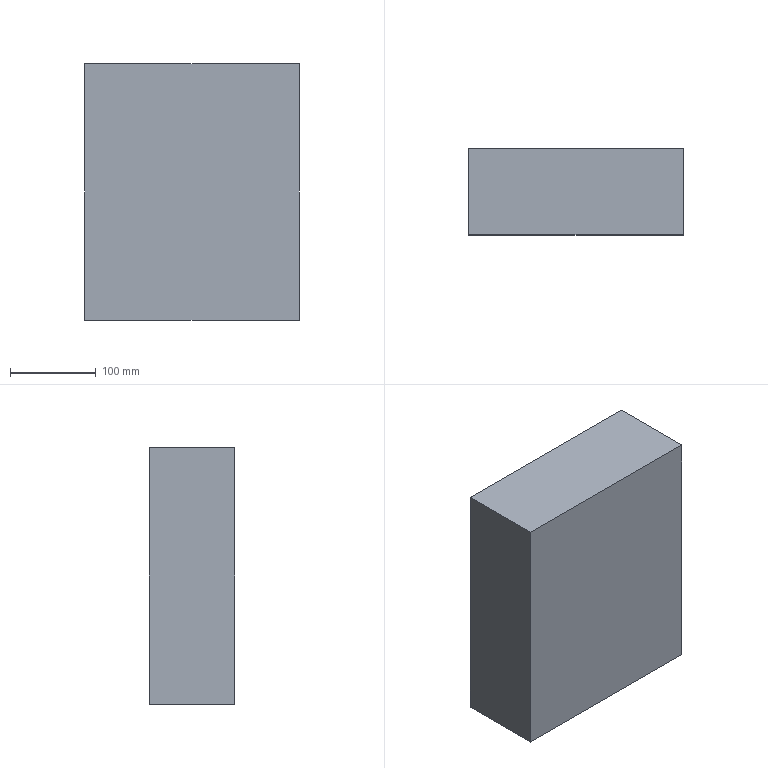Component | SolidWorks | InsectCollectionBox-1 | 1 solid | 11 faces | box 250 x 100 x 300 mm | volume 274138 mm3 | plane 11
build123d program:
from build123d import *

# Parameters (mm, degrees)
SKETCH1_W           = 300
SKETCH1_H           = 250
BOSS_EXTRUDE1_DEPTH = 100
SHELL1_T            = -1.5


with BuildPart() as part:
    # Sketch1 → Boss-Extrude1 (new body)
    with BuildSketch(Plane(origin=(0, 0, 0), x_dir=(1, 0, 0), z_dir=(0, 1, 0))):
        Rectangle(SKETCH1_W, SKETCH1_H)
    extrude(amount=BOSS_EXTRUDE1_DEPTH)

    # Shell1
    shell1_openings = [part.faces().sort_by_distance(p)[0] for p in [
        (0, 100, 0),
    ]]
    offset(amount=SHELL1_T, openings=shell1_openings, kind=Kind.INTERSECTION)


solid = part.part

# Placed as in the assembly
solid = solid.moved(Location((173.5, 1.5, 0), (0, 90, 0)))
STEP:
#1=COLOUR_RGB('',0.7922,0.8196,0.9333);
#2=FILL_AREA_STYLE_COLOUR('',#1);
#3=FILL_AREA_STYLE('',(#2));
#4=SURFACE_STYLE_FILL_AREA(#3);
#5=SURFACE_SIDE_STYLE('',(#4));
#6=SURFACE_STYLE_USAGE(.BOTH.,#5);
#7=PRESENTATION_STYLE_ASSIGNMENT((#6));
#8=CARTESIAN_POINT('',(11.752,0.05906,-5.906));
#9=VERTEX_POINT('',#8);
#10=CARTESIAN_POINT('',(1.909,0.05906,-5.906));
#11=VERTEX_POINT('',#10);
#12=CARTESIAN_POINT('',(1.909,0.05906,-5.906));
#13=DIRECTION('',(-1.,0.,0.));
#14=VECTOR('',#13,39.37);
#15=LINE('',#12,#14);
#16=EDGE_CURVE('',#9,#11,#15,.T.);
#17=ORIENTED_EDGE('',*,*,#16,.T.);
#18=CARTESIAN_POINT('',(1.909,3.996,-5.906));
#19=VERTEX_POINT('',#18);
#20=CARTESIAN_POINT('',(1.909,3.996,-5.906));
#21=DIRECTION('',(0.,-1.,0.));
#22=VECTOR('',#21,39.37);
#23=LINE('',#20,#22);
#24=EDGE_CURVE('',#19,#11,#23,.T.);
#25=ORIENTED_EDGE('',*,*,#24,.F.);
#26=CARTESIAN_POINT('',(11.752,3.996,-5.906));
#27=VERTEX_POINT('',#26);
#28=CARTESIAN_POINT('',(1.909,3.996,-5.906));
#29=DIRECTION('',(-1.,0.,0.));
#30=VECTOR('',#29,39.37);
#31=LINE('',#28,#30);
#32=EDGE_CURVE('',#27,#19,#31,.T.);
#33=ORIENTED_EDGE('',*,*,#32,.F.);
#34=CARTESIAN_POINT('',(11.752,3.996,-5.906));
#35=DIRECTION('',(0.,-1.,0.));
#36=VECTOR('',#35,39.37);
#37=LINE('',#34,#36);
#38=EDGE_CURVE('',#27,#9,#37,.T.);
#39=ORIENTED_EDGE('',*,*,#38,.T.);
#40=EDGE_LOOP('',(#17,#25,#33,#39));
#41=FACE_OUTER_BOUND('',#40,.T.);
#42=CARTESIAN_POINT('',(1.909,3.996,-5.906));
#43=DIRECTION('',(0.,0.,1.));
#44=DIRECTION('',(1.,0.,0.));
#45=AXIS2_PLACEMENT_3D('',#42,#43,#44);
#46=PLANE('',#45);
#47=ADVANCED_FACE('',(#41),#46,.F.);
#48=CARTESIAN_POINT('',(1.909,0.05906,5.906));
#49=VERTEX_POINT('',#48);
#50=CARTESIAN_POINT('',(1.909,0.05906,5.906));
#51=DIRECTION('',(0.,0.,1.));
#52=VECTOR('',#51,39.37);
#53=LINE('',#50,#52);
#54=EDGE_CURVE('',#11,#49,#53,.T.);
#55=ORIENTED_EDGE('',*,*,#54,.T.);
#56=CARTESIAN_POINT('',(1.909,3.996,5.906));
#57=VERTEX_POINT('',#56);
#58=CARTESIAN_POINT('',(1.909,3.996,5.906));
#59=DIRECTION('',(0.,-1.,0.));
#60=VECTOR('',#59,39.37);
#61=LINE('',#58,#60);
#62=EDGE_CURVE('',#57,#49,#61,.T.);
#63=ORIENTED_EDGE('',*,*,#62,.F.);
#64=CARTESIAN_POINT('',(1.909,3.996,5.906));
#65=DIRECTION('',(0.,0.,1.));
#66=VECTOR('',#65,39.37);
#67=LINE('',#64,#66);
#68=EDGE_CURVE('',#19,#57,#67,.T.);
#69=ORIENTED_EDGE('',*,*,#68,.F.);
#70=ORIENTED_EDGE('',*,*,#24,.T.);
#71=EDGE_LOOP('',(#55,#63,#69,#70));
#72=FACE_OUTER_BOUND('',#71,.T.);
#73=CARTESIAN_POINT('',(1.909,3.996,5.906));
#74=DIRECTION('',(1.,0.,0.));
#75=DIRECTION('',(0.,0.,-1.));
#76=AXIS2_PLACEMENT_3D('',#73,#74,#75);
#77=PLANE('',#76);
#78=ADVANCED_FACE('',(#72),#77,.F.);
#79=CARTESIAN_POINT('',(11.752,0.05906,5.906));
#80=VERTEX_POINT('',#79);
#81=CARTESIAN_POINT('',(1.909,0.05906,5.906));
#82=DIRECTION('',(1.,0.,0.));
#83=VECTOR('',#82,39.37);
#84=LINE('',#81,#83);
#85=EDGE_CURVE('',#49,#80,#84,.T.);
#86=ORIENTED_EDGE('',*,*,#85,.T.);
#87=CARTESIAN_POINT('',(11.752,3.996,5.906));
#88=VERTEX_POINT('',#87);
#89=CARTESIAN_POINT('',(11.752,3.996,5.906));
#90=DIRECTION('',(0.,-1.,0.));
#91=VECTOR('',#90,39.37);
#92=LINE('',#89,#91);
#93=EDGE_CURVE('',#88,#80,#92,.T.);
#94=ORIENTED_EDGE('',*,*,#93,.F.);
#95=CARTESIAN_POINT('',(1.909,3.996,5.906));
#96=DIRECTION('',(1.,0.,0.));
#97=VECTOR('',#96,39.37);
#98=LINE('',#95,#97);
#99=EDGE_CURVE('',#57,#88,#98,.T.);
#100=ORIENTED_EDGE('',*,*,#99,.F.);
#101=ORIENTED_EDGE('',*,*,#62,.T.);
#102=EDGE_LOOP('',(#86,#94,#100,#101));
#103=FACE_OUTER_BOUND('',#102,.T.);
#104=CARTESIAN_POINT('',(1.909,3.996,5.906));
#105=DIRECTION('',(0.,0.,-1.));
#106=DIRECTION('',(-1.,0.,0.));
#107=AXIS2_PLACEMENT_3D('',#104,#105,#106);
#108=PLANE('',#107);
#109=ADVANCED_FACE('',(#103),#108,.F.);
#110=CARTESIAN_POINT('',(11.752,0.05906,5.906));
#111=DIRECTION('',(0.,0.,-1.));
#112=VECTOR('',#111,39.37);
#113=LINE('',#110,#112);
#114=EDGE_CURVE('',#80,#9,#113,.T.);
#115=ORIENTED_EDGE('',*,*,#114,.T.);
#116=ORIENTED_EDGE('',*,*,#38,.F.);
#117=CARTESIAN_POINT('',(11.752,3.996,5.906));
#118=DIRECTION('',(0.,0.,-1.));
#119=VECTOR('',#118,39.37);
#120=LINE('',#117,#119);
#121=EDGE_CURVE('',#88,#27,#120,.T.);
#122=ORIENTED_EDGE('',*,*,#121,.F.);
#123=ORIENTED_EDGE('',*,*,#93,.T.);
#124=EDGE_LOOP('',(#115,#116,#122,#123));
#125=FACE_OUTER_BOUND('',#124,.T.);
#126=CARTESIAN_POINT('',(11.752,3.996,5.906));
#127=DIRECTION('',(-1.,0.,0.));
#128=DIRECTION('',(0.,0.,1.));
#129=AXIS2_PLACEMENT_3D('',#126,#127,#128);
#130=PLANE('',#129);
#131=ADVANCED_FACE('',(#125),#130,.F.);
#132=CARTESIAN_POINT('',(11.693,3.996,-5.846));
#133=VERTEX_POINT('',#132);
#134=CARTESIAN_POINT('',(1.969,3.996,-5.846));
#135=VERTEX_POINT('',#134);
#136=CARTESIAN_POINT('',(1.909,3.996,-5.846));
#137=DIRECTION('',(-1.,0.,0.));
#138=VECTOR('',#137,39.37);
#139=LINE('',#136,#138);
#140=EDGE_CURVE('',#133,#135,#139,.T.);
#141=ORIENTED_EDGE('',*,*,#140,.F.);
#142=CARTESIAN_POINT('',(11.693,3.996,5.846));
#143=VERTEX_POINT('',#142);
#144=CARTESIAN_POINT('',(11.693,3.996,5.906));
#145=DIRECTION('',(0.,0.,-1.));
#146=VECTOR('',#145,39.37);
#147=LINE('',#144,#146);
#148=EDGE_CURVE('',#143,#133,#147,.T.);
#149=ORIENTED_EDGE('',*,*,#148,.F.);
#150=CARTESIAN_POINT('',(1.969,3.996,5.846));
#151=VERTEX_POINT('',#150);
#152=CARTESIAN_POINT('',(1.909,3.996,5.846));
#153=DIRECTION('',(1.,0.,0.));
#154=VECTOR('',#153,39.37);
#155=LINE('',#152,#154);
#156=EDGE_CURVE('',#151,#143,#155,.T.);
#157=ORIENTED_EDGE('',*,*,#156,.F.);
#158=CARTESIAN_POINT('',(1.969,3.996,5.906));
#159=DIRECTION('',(0.,0.,1.));
#160=VECTOR('',#159,39.37);
#161=LINE('',#158,#160);
#162=EDGE_CURVE('',#135,#151,#161,.T.);
#163=ORIENTED_EDGE('',*,*,#162,.F.);
#164=EDGE_LOOP('',(#141,#149,#157,#163));
#165=FACE_BOUND('',#164,.T.);
#166=ORIENTED_EDGE('',*,*,#32,.T.);
#167=ORIENTED_EDGE('',*,*,#68,.T.);
#168=ORIENTED_EDGE('',*,*,#99,.T.);
#169=ORIENTED_EDGE('',*,*,#121,.T.);
#170=EDGE_LOOP('',(#166,#167,#168,#169));
#171=FACE_OUTER_BOUND('',#170,.T.);
#172=CARTESIAN_POINT('',(6.831,3.996,0.));
#173=DIRECTION('',(0.,1.,0.));
#174=DIRECTION('',(1.,0.,0.));
#175=AXIS2_PLACEMENT_3D('',#172,#173,#174);
#176=PLANE('',#175);
#177=ADVANCED_FACE('',(#165,#171),#176,.T.);
#178=ORIENTED_EDGE('',*,*,#16,.F.);
#179=ORIENTED_EDGE('',*,*,#114,.F.);
#180=ORIENTED_EDGE('',*,*,#85,.F.);
#181=ORIENTED_EDGE('',*,*,#54,.F.);
#182=EDGE_LOOP('',(#178,#179,#180,#181));
#183=FACE_OUTER_BOUND('',#182,.T.);
#184=CARTESIAN_POINT('',(6.831,0.05906,0.));
#185=DIRECTION('',(0.,1.,0.));
#186=DIRECTION('',(1.,0.,0.));
#187=AXIS2_PLACEMENT_3D('',#184,#185,#186);
#188=PLANE('',#187);
#189=ADVANCED_FACE('',(#183),#188,.F.);
#190=CARTESIAN_POINT('',(11.693,0.1181,-5.846));
#191=VERTEX_POINT('',#190);
#192=CARTESIAN_POINT('',(1.969,0.1181,-5.846));
#193=VERTEX_POINT('',#192);
#194=CARTESIAN_POINT('',(1.909,0.1181,-5.846));
#195=DIRECTION('',(-1.,0.,0.));
#196=VECTOR('',#195,39.37);
#197=LINE('',#194,#196);
#198=EDGE_CURVE('',#191,#193,#197,.T.);
#199=ORIENTED_EDGE('',*,*,#198,.F.);
#200=CARTESIAN_POINT('',(11.693,3.996,-5.846));
#201=DIRECTION('',(0.,-1.,0.));
#202=VECTOR('',#201,39.37);
#203=LINE('',#200,#202);
#204=EDGE_CURVE('',#133,#191,#203,.T.);
#205=ORIENTED_EDGE('',*,*,#204,.F.);
#206=ORIENTED_EDGE('',*,*,#140,.T.);
#207=CARTESIAN_POINT('',(1.969,3.996,-5.846));
#208=DIRECTION('',(0.,-1.,0.));
#209=VECTOR('',#208,39.37);
#210=LINE('',#207,#209);
#211=EDGE_CURVE('',#135,#193,#210,.T.);
#212=ORIENTED_EDGE('',*,*,#211,.T.);
#213=EDGE_LOOP('',(#199,#205,#206,#212));
#214=FACE_OUTER_BOUND('',#213,.T.);
#215=CARTESIAN_POINT('',(1.909,3.996,-5.846));
#216=DIRECTION('',(0.,0.,1.));
#217=DIRECTION('',(1.,0.,0.));
#218=AXIS2_PLACEMENT_3D('',#215,#216,#217);
#219=PLANE('',#218);
#220=ADVANCED_FACE('',(#214),#219,.T.);
#221=CARTESIAN_POINT('',(1.969,0.1181,5.846));
#222=VERTEX_POINT('',#221);
#223=CARTESIAN_POINT('',(1.969,0.1181,5.906));
#224=DIRECTION('',(0.,0.,1.));
#225=VECTOR('',#224,39.37);
#226=LINE('',#223,#225);
#227=EDGE_CURVE('',#193,#222,#226,.T.);
#228=ORIENTED_EDGE('',*,*,#227,.F.);
#229=ORIENTED_EDGE('',*,*,#211,.F.);
#230=ORIENTED_EDGE('',*,*,#162,.T.);
#231=CARTESIAN_POINT('',(1.969,3.996,5.846));
#232=DIRECTION('',(0.,-1.,0.));
#233=VECTOR('',#232,39.37);
#234=LINE('',#231,#233);
#235=EDGE_CURVE('',#151,#222,#234,.T.);
#236=ORIENTED_EDGE('',*,*,#235,.T.);
#237=EDGE_LOOP('',(#228,#229,#230,#236));
#238=FACE_OUTER_BOUND('',#237,.T.);
#239=CARTESIAN_POINT('',(1.969,3.996,5.906));
#240=DIRECTION('',(1.,0.,0.));
#241=DIRECTION('',(0.,0.,-1.));
#242=AXIS2_PLACEMENT_3D('',#239,#240,#241);
#243=PLANE('',#242);
#244=ADVANCED_FACE('',(#238),#243,.T.);
#245=CARTESIAN_POINT('',(11.693,0.1181,5.846));
#246=VERTEX_POINT('',#245);
#247=CARTESIAN_POINT('',(1.909,0.1181,5.846));
#248=DIRECTION('',(1.,0.,0.));
#249=VECTOR('',#248,39.37);
#250=LINE('',#247,#249);
#251=EDGE_CURVE('',#222,#246,#250,.T.);
#252=ORIENTED_EDGE('',*,*,#251,.F.);
#253=ORIENTED_EDGE('',*,*,#235,.F.);
#254=ORIENTED_EDGE('',*,*,#156,.T.);
#255=CARTESIAN_POINT('',(11.693,3.996,5.846));
#256=DIRECTION('',(0.,-1.,0.));
#257=VECTOR('',#256,39.37);
#258=LINE('',#255,#257);
#259=EDGE_CURVE('',#143,#246,#258,.T.);
#260=ORIENTED_EDGE('',*,*,#259,.T.);
#261=EDGE_LOOP('',(#252,#253,#254,#260));
#262=FACE_OUTER_BOUND('',#261,.T.);
#263=CARTESIAN_POINT('',(1.909,3.996,5.846));
#264=DIRECTION('',(0.,0.,-1.));
#265=DIRECTION('',(-1.,0.,0.));
#266=AXIS2_PLACEMENT_3D('',#263,#264,#265);
#267=PLANE('',#266);
#268=ADVANCED_FACE('',(#262),#267,.T.);
#269=CARTESIAN_POINT('',(11.693,0.1181,5.906));
#270=DIRECTION('',(0.,0.,-1.));
#271=VECTOR('',#270,39.37);
#272=LINE('',#269,#271);
#273=EDGE_CURVE('',#246,#191,#272,.T.);
#274=ORIENTED_EDGE('',*,*,#273,.F.);
#275=ORIENTED_EDGE('',*,*,#259,.F.);
#276=ORIENTED_EDGE('',*,*,#148,.T.);
#277=ORIENTED_EDGE('',*,*,#204,.T.);
#278=EDGE_LOOP('',(#274,#275,#276,#277));
#279=FACE_OUTER_BOUND('',#278,.T.);
#280=CARTESIAN_POINT('',(11.693,3.996,5.906));
#281=DIRECTION('',(-1.,0.,0.));
#282=DIRECTION('',(0.,0.,1.));
#283=AXIS2_PLACEMENT_3D('',#280,#281,#282);
#284=PLANE('',#283);
#285=ADVANCED_FACE('',(#279),#284,.T.);
#286=ORIENTED_EDGE('',*,*,#198,.T.);
#287=ORIENTED_EDGE('',*,*,#227,.T.);
#288=ORIENTED_EDGE('',*,*,#251,.T.);
#289=ORIENTED_EDGE('',*,*,#273,.T.);
#290=EDGE_LOOP('',(#286,#287,#288,#289));
#291=FACE_OUTER_BOUND('',#290,.T.);
#292=CARTESIAN_POINT('',(6.831,0.1181,0.));
#293=DIRECTION('',(0.,1.,0.));
#294=DIRECTION('',(1.,0.,0.));
#295=AXIS2_PLACEMENT_3D('',#292,#293,#294);
#296=PLANE('',#295);
#297=ADVANCED_FACE('',(#291),#296,.T.);
#298=CLOSED_SHELL('',(#47,#78,#109,#131,#177,#189,#220,#244,#268,#285,#297));
#299=MANIFOLD_SOLID_BREP('',#298);
#300=STYLED_ITEM('',(#7),#299);
#301=PRESENTATION_LAYER_ASSIGNMENT('','',(#300));
#302=(LENGTH_UNIT()NAMED_UNIT(*)SI_UNIT($,.METRE.));
#303=LENGTH_MEASURE_WITH_UNIT(LENGTH_MEASURE(0.0254),#302);
#304=DIMENSIONAL_EXPONENTS(1.,0.,0.,0.,0.,0.,0.);
#305=(CONVERSION_BASED_UNIT('',#303)LENGTH_UNIT()NAMED_UNIT(#304));
#306=UNCERTAINTY_MEASURE_WITH_UNIT(LENGTH_MEASURE(0.00001),#305,'','');
#307=(NAMED_UNIT(*)PLANE_ANGLE_UNIT()SI_UNIT($,.RADIAN.));
#308=(NAMED_UNIT(*)SI_UNIT($,.STERADIAN.)SOLID_ANGLE_UNIT());
#309=(GEOMETRIC_REPRESENTATION_CONTEXT(3)GLOBAL_UNCERTAINTY_ASSIGNED_CONTEXT((#306))GLOBAL_UNIT_ASSIGNED_CONTEXT((#305,#307,#308))REPRESENTATION_CONTEXT('',''));
#310=MECHANICAL_DESIGN_GEOMETRIC_PRESENTATION_REPRESENTATION('',(#300),#309);
#311=CARTESIAN_POINT('',(0.,0.,0.));
#312=DIRECTION('',(0.,0.,1.));
#313=DIRECTION('',(1.,0.,0.));
#314=AXIS2_PLACEMENT_3D('',#311,#312,#313);
#315=(LENGTH_UNIT()NAMED_UNIT(*)SI_UNIT($,.METRE.));
#316=LENGTH_MEASURE_WITH_UNIT(LENGTH_MEASURE(0.0254),#315);
#317=DIMENSIONAL_EXPONENTS(1.,0.,0.,0.,0.,0.,0.);
#318=(CONVERSION_BASED_UNIT('',#316)LENGTH_UNIT()NAMED_UNIT(#317));
#319=UNCERTAINTY_MEASURE_WITH_UNIT(LENGTH_MEASURE(0.00001),#318,'','');
#320=(NAMED_UNIT(*)PLANE_ANGLE_UNIT()SI_UNIT($,.RADIAN.));
#321=(NAMED_UNIT(*)SI_UNIT($,.STERADIAN.)SOLID_ANGLE_UNIT());
#322=(GEOMETRIC_REPRESENTATION_CONTEXT(3)GLOBAL_UNCERTAINTY_ASSIGNED_CONTEXT((#319))GLOBAL_UNIT_ASSIGNED_CONTEXT((#318,#320,#321))REPRESENTATION_CONTEXT('',''));
#323=ADVANCED_BREP_SHAPE_REPRESENTATION('',(#299,#314),#322);